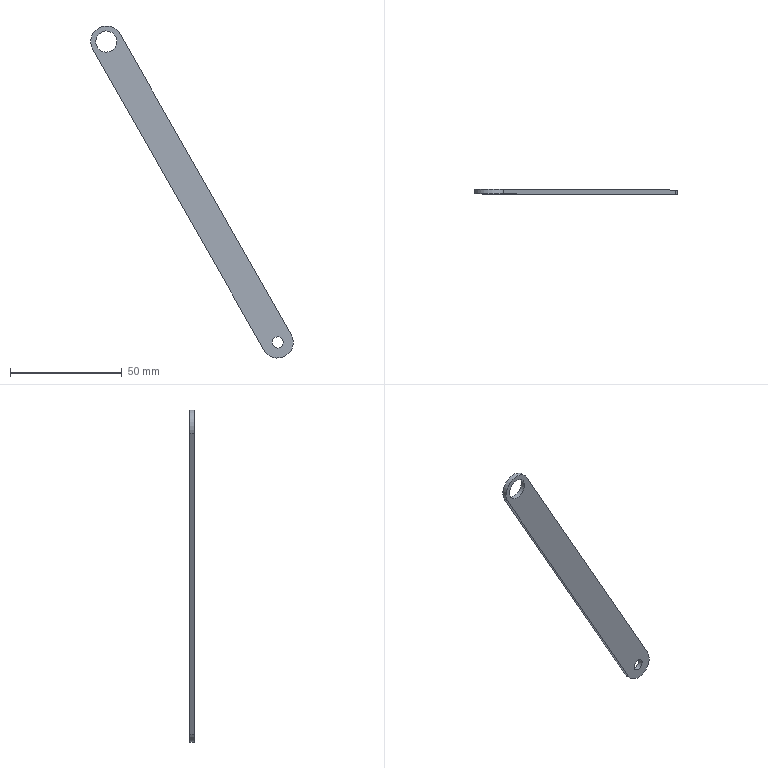Component | NX | 8 | 1 solid | 8 faces | box 90.7 x 2 x 148.69 mm | volume 4467 mm3 | cylinder 4 | plane 4 | commonest cylinder face diameters 14 x2 5 x1 9.5 x1
STEP:
#1=CARTESIAN_POINT('',(0.,0.,0.));
#2=DIRECTION('',(0.,0.,1.));
#3=DIRECTION('',(1.,0.,0.));
#4=AXIS2_PLACEMENT_3D('',#1,#2,#3);
#5=CARTESIAN_POINT('',(-289.091,186.249,-214.872));
#6=VERTEX_POINT('',#5);
#7=CARTESIAN_POINT('',(-276.925,186.249,-207.944));
#8=VERTEX_POINT('',#7);
#9=CARTESIAN_POINT('',(-283.008,186.249,-211.408));
#10=DIRECTION('',(0.,-1.,0.));
#11=DIRECTION('',(0.4948,0.,-0.869));
#12=AXIS2_PLACEMENT_3D('',#9,#10,#11);
#13=CIRCLE('',#12,7.);
#14=CARTESIAN_POINT('',(-283.008,184.249,-211.408));
#15=DIRECTION('',(0.,1.,0.));
#16=DIRECTION('',(0.4948,0.,-0.869));
#17=AXIS2_PLACEMENT_3D('',#14,#15,#16);
#18=CYLINDRICAL_SURFACE('',#17,7.);
#19=CARTESIAN_POINT('',(6.283,2.));
#20=DIRECTION('',(-1.,0.));
#21=VECTOR('',#20,1.);
#22=LINE('',#19,#21);
#23=(GEOMETRIC_REPRESENTATION_CONTEXT(2)PARAMETRIC_REPRESENTATION_CONTEXT()REPRESENTATION_CONTEXT('',''));
#24=DEFINITIONAL_REPRESENTATION('',(#22),#23);
#25=PCURVE('',#18,#24);
#26=CARTESIAN_POINT('',(-283.008,186.249,-211.408));
#27=DIRECTION('',(0.,-1.,0.));
#28=DIRECTION('',(-0.4948,0.,0.869));
#29=AXIS2_PLACEMENT_3D('',#26,#27,#28);
#30=PLANE('',#29);
#31=CARTESIAN_POINT('',(0.,0.));
#32=DIRECTION('',(-1.,0.));
#33=AXIS2_PLACEMENT_2D('',#31,#32);
#34=CIRCLE('',#33,7.);
#35=(GEOMETRIC_REPRESENTATION_CONTEXT(2)PARAMETRIC_REPRESENTATION_CONTEXT()REPRESENTATION_CONTEXT('',''));
#36=DEFINITIONAL_REPRESENTATION('',(#34),#35);
#37=PCURVE('',#30,#36);
#38=SURFACE_CURVE('',#13,(#25,#37),.PCURVE_S1.);
#39=EDGE_CURVE('',#6,#8,#38,.T.);
#40=ORIENTED_EDGE('',*,*,#39,.T.);
#41=CARTESIAN_POINT('',(-276.925,184.249,-207.944));
#42=VERTEX_POINT('',#41);
#43=CARTESIAN_POINT('',(-276.925,184.249,-207.944));
#44=DIRECTION('',(0.,1.,0.));
#45=VECTOR('',#44,1.);
#46=LINE('',#43,#45);
#47=CARTESIAN_POINT('',(-1.571,0.));
#48=DIRECTION('',(0.,1.));
#49=VECTOR('',#48,1.);
#50=LINE('',#47,#49);
#51=(GEOMETRIC_REPRESENTATION_CONTEXT(2)PARAMETRIC_REPRESENTATION_CONTEXT()REPRESENTATION_CONTEXT('',''));
#52=DEFINITIONAL_REPRESENTATION('',(#50),#51);
#53=PCURVE('',#18,#52);
#54=CARTESIAN_POINT('',(-276.925,184.249,-207.944));
#55=DIRECTION('',(-0.869,0.,-0.4948));
#56=DIRECTION('',(0.,-1.,0.));
#57=AXIS2_PLACEMENT_3D('',#54,#55,#56);
#58=PLANE('',#57);
#59=CARTESIAN_POINT('',(0.,-0.));
#60=DIRECTION('',(-1.,0.));
#61=VECTOR('',#60,1.);
#62=LINE('',#59,#61);
#63=(GEOMETRIC_REPRESENTATION_CONTEXT(2)PARAMETRIC_REPRESENTATION_CONTEXT()REPRESENTATION_CONTEXT('',''));
#64=DEFINITIONAL_REPRESENTATION('',(#62),#63);
#65=PCURVE('',#58,#64);
#66=SURFACE_CURVE('',#46,(#53,#65),.PCURVE_S1.);
#67=EDGE_CURVE('',#42,#8,#66,.T.);
#68=ORIENTED_EDGE('',*,*,#67,.F.);
#69=CARTESIAN_POINT('',(-289.091,184.249,-214.872));
#70=VERTEX_POINT('',#69);
#71=CARTESIAN_POINT('',(-283.008,184.249,-211.408));
#72=DIRECTION('',(0.,-1.,0.));
#73=DIRECTION('',(0.4948,0.,-0.869));
#74=AXIS2_PLACEMENT_3D('',#71,#72,#73);
#75=CIRCLE('',#74,7.);
#76=CARTESIAN_POINT('',(6.283,0.));
#77=DIRECTION('',(-1.,0.));
#78=VECTOR('',#77,1.);
#79=LINE('',#76,#78);
#80=(GEOMETRIC_REPRESENTATION_CONTEXT(2)PARAMETRIC_REPRESENTATION_CONTEXT()REPRESENTATION_CONTEXT('',''));
#81=DEFINITIONAL_REPRESENTATION('',(#79),#80);
#82=PCURVE('',#18,#81);
#83=CARTESIAN_POINT('',(-283.008,184.249,-211.408));
#84=DIRECTION('',(0.,-1.,0.));
#85=DIRECTION('',(-0.4948,0.,0.869));
#86=AXIS2_PLACEMENT_3D('',#83,#84,#85);
#87=PLANE('',#86);
#88=CARTESIAN_POINT('',(0.,0.));
#89=DIRECTION('',(-1.,0.));
#90=AXIS2_PLACEMENT_2D('',#88,#89);
#91=CIRCLE('',#90,7.);
#92=(GEOMETRIC_REPRESENTATION_CONTEXT(2)PARAMETRIC_REPRESENTATION_CONTEXT()REPRESENTATION_CONTEXT('',''));
#93=DEFINITIONAL_REPRESENTATION('',(#91),#92);
#94=PCURVE('',#87,#93);
#95=SURFACE_CURVE('',#75,(#82,#94),.PCURVE_S1.);
#96=EDGE_CURVE('',#70,#42,#95,.T.);
#97=ORIENTED_EDGE('',*,*,#96,.F.);
#98=CARTESIAN_POINT('',(-289.091,184.249,-214.872));
#99=DIRECTION('',(0.,1.,0.));
#100=VECTOR('',#99,1.);
#101=LINE('',#98,#100);
#102=CARTESIAN_POINT('',(1.571,0.));
#103=DIRECTION('',(0.,1.));
#104=VECTOR('',#103,1.);
#105=LINE('',#102,#104);
#106=(GEOMETRIC_REPRESENTATION_CONTEXT(2)PARAMETRIC_REPRESENTATION_CONTEXT()REPRESENTATION_CONTEXT('',''));
#107=DEFINITIONAL_REPRESENTATION('',(#105),#106);
#108=PCURVE('',#18,#107);
#109=CARTESIAN_POINT('',(-365.788,184.249,-80.178));
#110=DIRECTION('',(0.869,0.,0.4948));
#111=DIRECTION('',(0.,1.,0.));
#112=AXIS2_PLACEMENT_3D('',#109,#110,#111);
#113=PLANE('',#112);
#114=CARTESIAN_POINT('',(0.,-155.));
#115=DIRECTION('',(1.,0.));
#116=VECTOR('',#115,1.);
#117=LINE('',#114,#116);
#118=(GEOMETRIC_REPRESENTATION_CONTEXT(2)PARAMETRIC_REPRESENTATION_CONTEXT()REPRESENTATION_CONTEXT('',''));
#119=DEFINITIONAL_REPRESENTATION('',(#117),#118);
#120=PCURVE('',#113,#119);
#121=SURFACE_CURVE('',#101,(#108,#120),.PCURVE_S1.);
#122=EDGE_CURVE('',#70,#6,#121,.T.);
#123=ORIENTED_EDGE('',*,*,#122,.T.);
#124=EDGE_LOOP('',(#40,#68,#97,#123));
#125=FACE_BOUND('',#124,.T.);
#126=ADVANCED_FACE('',(#125),#18,.T.);
#127=CARTESIAN_POINT('',(-353.622,186.249,-73.25));
#128=VERTEX_POINT('',#127);
#129=CARTESIAN_POINT('',(-276.925,186.249,-207.944));
#130=DIRECTION('',(-0.4948,0.,0.869));
#131=VECTOR('',#130,1.);
#132=LINE('',#129,#131);
#133=CARTESIAN_POINT('',(-2.,0.));
#134=DIRECTION('',(0.,1.));
#135=VECTOR('',#134,1.);
#136=LINE('',#133,#135);
#137=(GEOMETRIC_REPRESENTATION_CONTEXT(2)PARAMETRIC_REPRESENTATION_CONTEXT()REPRESENTATION_CONTEXT('',''));
#138=DEFINITIONAL_REPRESENTATION('',(#136),#137);
#139=PCURVE('',#58,#138);
#140=CARTESIAN_POINT('',(0.,-7.));
#141=DIRECTION('',(1.,0.));
#142=VECTOR('',#141,1.);
#143=LINE('',#140,#142);
#144=(GEOMETRIC_REPRESENTATION_CONTEXT(2)PARAMETRIC_REPRESENTATION_CONTEXT()REPRESENTATION_CONTEXT('',''));
#145=DEFINITIONAL_REPRESENTATION('',(#143),#144);
#146=PCURVE('',#30,#145);
#147=SURFACE_CURVE('',#132,(#139,#146),.PCURVE_S1.);
#148=EDGE_CURVE('',#8,#128,#147,.T.);
#149=ORIENTED_EDGE('',*,*,#148,.T.);
#150=CARTESIAN_POINT('',(-353.622,184.249,-73.25));
#151=VERTEX_POINT('',#150);
#152=CARTESIAN_POINT('',(-353.622,184.249,-73.25));
#153=DIRECTION('',(0.,1.,0.));
#154=VECTOR('',#153,1.);
#155=LINE('',#152,#154);
#156=CARTESIAN_POINT('',(0.,155.));
#157=DIRECTION('',(-1.,0.));
#158=VECTOR('',#157,1.);
#159=LINE('',#156,#158);
#160=(GEOMETRIC_REPRESENTATION_CONTEXT(2)PARAMETRIC_REPRESENTATION_CONTEXT()REPRESENTATION_CONTEXT('',''));
#161=DEFINITIONAL_REPRESENTATION('',(#159),#160);
#162=PCURVE('',#58,#161);
#163=CARTESIAN_POINT('',(-359.705,184.249,-76.714));
#164=DIRECTION('',(0.,1.,0.));
#165=DIRECTION('',(0.4948,0.,-0.869));
#166=AXIS2_PLACEMENT_3D('',#163,#164,#165);
#167=CYLINDRICAL_SURFACE('',#166,7.);
#168=CARTESIAN_POINT('',(4.712,0.));
#169=DIRECTION('',(0.,1.));
#170=VECTOR('',#169,1.);
#171=LINE('',#168,#170);
#172=(GEOMETRIC_REPRESENTATION_CONTEXT(2)PARAMETRIC_REPRESENTATION_CONTEXT()REPRESENTATION_CONTEXT('',''));
#173=DEFINITIONAL_REPRESENTATION('',(#171),#172);
#174=PCURVE('',#167,#173);
#175=SURFACE_CURVE('',#155,(#162,#174),.PCURVE_S1.);
#176=EDGE_CURVE('',#151,#128,#175,.T.);
#177=ORIENTED_EDGE('',*,*,#176,.F.);
#178=CARTESIAN_POINT('',(-276.925,184.249,-207.944));
#179=DIRECTION('',(-0.4948,0.,0.869));
#180=VECTOR('',#179,1.);
#181=LINE('',#178,#180);
#182=CARTESIAN_POINT('',(0.,0.));
#183=DIRECTION('',(0.,1.));
#184=VECTOR('',#183,1.);
#185=LINE('',#182,#184);
#186=(GEOMETRIC_REPRESENTATION_CONTEXT(2)PARAMETRIC_REPRESENTATION_CONTEXT()REPRESENTATION_CONTEXT('',''));
#187=DEFINITIONAL_REPRESENTATION('',(#185),#186);
#188=PCURVE('',#58,#187);
#189=CARTESIAN_POINT('',(0.,-7.));
#190=DIRECTION('',(1.,0.));
#191=VECTOR('',#190,1.);
#192=LINE('',#189,#191);
#193=(GEOMETRIC_REPRESENTATION_CONTEXT(2)PARAMETRIC_REPRESENTATION_CONTEXT()REPRESENTATION_CONTEXT('',''));
#194=DEFINITIONAL_REPRESENTATION('',(#192),#193);
#195=PCURVE('',#87,#194);
#196=SURFACE_CURVE('',#181,(#188,#195),.PCURVE_S1.);
#197=EDGE_CURVE('',#42,#151,#196,.T.);
#198=ORIENTED_EDGE('',*,*,#197,.F.);
#199=ORIENTED_EDGE('',*,*,#67,.T.);
#200=EDGE_LOOP('',(#149,#177,#198,#199));
#201=FACE_BOUND('',#200,.T.);
#202=ADVANCED_FACE('',(#201),#58,.F.);
#203=CARTESIAN_POINT('',(-365.788,186.249,-80.178));
#204=VERTEX_POINT('',#203);
#205=CARTESIAN_POINT('',(-359.705,186.249,-76.714));
#206=DIRECTION('',(0.,-1.,0.));
#207=DIRECTION('',(0.4948,0.,-0.869));
#208=AXIS2_PLACEMENT_3D('',#205,#206,#207);
#209=CIRCLE('',#208,7.);
#210=CARTESIAN_POINT('',(6.283,2.));
#211=DIRECTION('',(-1.,0.));
#212=VECTOR('',#211,1.);
#213=LINE('',#210,#212);
#214=(GEOMETRIC_REPRESENTATION_CONTEXT(2)PARAMETRIC_REPRESENTATION_CONTEXT()REPRESENTATION_CONTEXT('',''));
#215=DEFINITIONAL_REPRESENTATION('',(#213),#214);
#216=PCURVE('',#167,#215);
#217=CARTESIAN_POINT('',(155.,0.));
#218=DIRECTION('',(-1.,-0.));
#219=AXIS2_PLACEMENT_2D('',#217,#218);
#220=CIRCLE('',#219,7.);
#221=(GEOMETRIC_REPRESENTATION_CONTEXT(2)PARAMETRIC_REPRESENTATION_CONTEXT()REPRESENTATION_CONTEXT('',''));
#222=DEFINITIONAL_REPRESENTATION('',(#220),#221);
#223=PCURVE('',#30,#222);
#224=SURFACE_CURVE('',#209,(#216,#223),.PCURVE_S1.);
#225=EDGE_CURVE('',#128,#204,#224,.T.);
#226=ORIENTED_EDGE('',*,*,#225,.T.);
#227=CARTESIAN_POINT('',(-365.788,184.249,-80.178));
#228=VERTEX_POINT('',#227);
#229=CARTESIAN_POINT('',(-365.788,184.249,-80.178));
#230=DIRECTION('',(0.,1.,0.));
#231=VECTOR('',#230,1.);
#232=LINE('',#229,#231);
#233=CARTESIAN_POINT('',(1.571,0.));
#234=DIRECTION('',(0.,1.));
#235=VECTOR('',#234,1.);
#236=LINE('',#233,#235);
#237=(GEOMETRIC_REPRESENTATION_CONTEXT(2)PARAMETRIC_REPRESENTATION_CONTEXT()REPRESENTATION_CONTEXT('',''));
#238=DEFINITIONAL_REPRESENTATION('',(#236),#237);
#239=PCURVE('',#167,#238);
#240=CARTESIAN_POINT('',(0.,0.));
#241=DIRECTION('',(1.,0.));
#242=VECTOR('',#241,1.);
#243=LINE('',#240,#242);
#244=(GEOMETRIC_REPRESENTATION_CONTEXT(2)PARAMETRIC_REPRESENTATION_CONTEXT()REPRESENTATION_CONTEXT('',''));
#245=DEFINITIONAL_REPRESENTATION('',(#243),#244);
#246=PCURVE('',#113,#245);
#247=SURFACE_CURVE('',#232,(#239,#246),.PCURVE_S1.);
#248=EDGE_CURVE('',#228,#204,#247,.T.);
#249=ORIENTED_EDGE('',*,*,#248,.F.);
#250=CARTESIAN_POINT('',(-359.705,184.249,-76.714));
#251=DIRECTION('',(0.,-1.,0.));
#252=DIRECTION('',(0.4948,0.,-0.869));
#253=AXIS2_PLACEMENT_3D('',#250,#251,#252);
#254=CIRCLE('',#253,7.);
#255=CARTESIAN_POINT('',(6.283,0.));
#256=DIRECTION('',(-1.,0.));
#257=VECTOR('',#256,1.);
#258=LINE('',#255,#257);
#259=(GEOMETRIC_REPRESENTATION_CONTEXT(2)PARAMETRIC_REPRESENTATION_CONTEXT()REPRESENTATION_CONTEXT('',''));
#260=DEFINITIONAL_REPRESENTATION('',(#258),#259);
#261=PCURVE('',#167,#260);
#262=CARTESIAN_POINT('',(155.,0.));
#263=DIRECTION('',(-1.,-0.));
#264=AXIS2_PLACEMENT_2D('',#262,#263);
#265=CIRCLE('',#264,7.);
#266=(GEOMETRIC_REPRESENTATION_CONTEXT(2)PARAMETRIC_REPRESENTATION_CONTEXT()REPRESENTATION_CONTEXT('',''));
#267=DEFINITIONAL_REPRESENTATION('',(#265),#266);
#268=PCURVE('',#87,#267);
#269=SURFACE_CURVE('',#254,(#261,#268),.PCURVE_S1.);
#270=EDGE_CURVE('',#151,#228,#269,.T.);
#271=ORIENTED_EDGE('',*,*,#270,.F.);
#272=ORIENTED_EDGE('',*,*,#176,.T.);
#273=EDGE_LOOP('',(#226,#249,#271,#272));
#274=FACE_BOUND('',#273,.T.);
#275=ADVANCED_FACE('',(#274),#167,.T.);
#276=CARTESIAN_POINT('',(-284.245,184.249,-209.236));
#277=VERTEX_POINT('',#276);
#278=CARTESIAN_POINT('',(-283.008,184.249,-211.408));
#279=DIRECTION('',(0.,-1.,0.));
#280=DIRECTION('',(-0.4948,0.,0.869));
#281=AXIS2_PLACEMENT_3D('',#278,#279,#280);
#282=CIRCLE('',#281,2.5);
#283=CARTESIAN_POINT('',(-283.008,184.249,-211.408));
#284=DIRECTION('',(0.,1.,0.));
#285=DIRECTION('',(0.4948,0.,-0.869));
#286=AXIS2_PLACEMENT_3D('',#283,#284,#285);
#287=CYLINDRICAL_SURFACE('',#286,2.5);
#288=CARTESIAN_POINT('',(9.425,0.));
#289=DIRECTION('',(-1.,0.));
#290=VECTOR('',#289,1.);
#291=LINE('',#288,#290);
#292=(GEOMETRIC_REPRESENTATION_CONTEXT(2)PARAMETRIC_REPRESENTATION_CONTEXT()REPRESENTATION_CONTEXT('',''));
#293=DEFINITIONAL_REPRESENTATION('',(#291),#292);
#294=PCURVE('',#287,#293);
#295=CARTESIAN_POINT('',(0.,0.));
#296=DIRECTION('',(1.,0.));
#297=AXIS2_PLACEMENT_2D('',#295,#296);
#298=CIRCLE('',#297,2.5);
#299=(GEOMETRIC_REPRESENTATION_CONTEXT(2)PARAMETRIC_REPRESENTATION_CONTEXT()REPRESENTATION_CONTEXT('',''));
#300=DEFINITIONAL_REPRESENTATION('',(#298),#299);
#301=PCURVE('',#87,#300);
#302=SURFACE_CURVE('',#282,(#294,#301),.PCURVE_S1.);
#303=EDGE_CURVE('',#277,#277,#302,.T.);
#304=ORIENTED_EDGE('',*,*,#303,.F.);
#305=CARTESIAN_POINT('',(-284.245,186.249,-209.236));
#306=VERTEX_POINT('',#305);
#307=CARTESIAN_POINT('',(-284.245,184.249,-209.236));
#308=CARTESIAN_POINT('',(-284.245,186.249,-209.236));
#309=B_SPLINE_CURVE_WITH_KNOTS('',1,(#307,#308),.UNSPECIFIED.,.F.,.F.,(2,2),(0.,2.),.PIECEWISE_BEZIER_KNOTS.);
#310=CARTESIAN_POINT('',(9.425,0.));
#311=DIRECTION('',(0.,1.));
#312=VECTOR('',#311,1.);
#313=LINE('',#310,#312);
#314=(GEOMETRIC_REPRESENTATION_CONTEXT(2)PARAMETRIC_REPRESENTATION_CONTEXT()REPRESENTATION_CONTEXT('',''));
#315=DEFINITIONAL_REPRESENTATION('',(#313),#314);
#316=PCURVE('',#287,#315);
#317=CARTESIAN_POINT('',(3.142,0.));
#318=DIRECTION('',(0.,1.));
#319=VECTOR('',#318,1.);
#320=LINE('',#317,#319);
#321=(GEOMETRIC_REPRESENTATION_CONTEXT(2)PARAMETRIC_REPRESENTATION_CONTEXT()REPRESENTATION_CONTEXT('',''));
#322=DEFINITIONAL_REPRESENTATION('',(#320),#321);
#323=PCURVE('',#287,#322);
#324=SEAM_CURVE('',#309,(#316,#323),.PCURVE_S1.);
#325=EDGE_CURVE('',#277,#306,#324,.T.);
#326=ORIENTED_EDGE('',*,*,#325,.T.);
#327=CARTESIAN_POINT('',(-283.008,186.249,-211.408));
#328=DIRECTION('',(0.,-1.,0.));
#329=DIRECTION('',(-0.4948,0.,0.869));
#330=AXIS2_PLACEMENT_3D('',#327,#328,#329);
#331=CIRCLE('',#330,2.5);
#332=CARTESIAN_POINT('',(9.425,2.));
#333=DIRECTION('',(-1.,0.));
#334=VECTOR('',#333,1.);
#335=LINE('',#332,#334);
#336=(GEOMETRIC_REPRESENTATION_CONTEXT(2)PARAMETRIC_REPRESENTATION_CONTEXT()REPRESENTATION_CONTEXT('',''));
#337=DEFINITIONAL_REPRESENTATION('',(#335),#336);
#338=PCURVE('',#287,#337);
#339=CARTESIAN_POINT('',(0.,0.));
#340=DIRECTION('',(1.,0.));
#341=AXIS2_PLACEMENT_2D('',#339,#340);
#342=CIRCLE('',#341,2.5);
#343=(GEOMETRIC_REPRESENTATION_CONTEXT(2)PARAMETRIC_REPRESENTATION_CONTEXT()REPRESENTATION_CONTEXT('',''));
#344=DEFINITIONAL_REPRESENTATION('',(#342),#343);
#345=PCURVE('',#30,#344);
#346=SURFACE_CURVE('',#331,(#338,#345),.PCURVE_S1.);
#347=EDGE_CURVE('',#306,#306,#346,.T.);
#348=ORIENTED_EDGE('',*,*,#347,.T.);
#349=ORIENTED_EDGE('',*,*,#325,.F.);
#350=EDGE_LOOP('',(#304,#326,#348,#349));
#351=FACE_BOUND('',#350,.F.);
#352=ADVANCED_FACE('',(#351),#287,.F.);
#353=CARTESIAN_POINT('',(-365.788,186.249,-80.178));
#354=DIRECTION('',(0.4948,0.,-0.869));
#355=VECTOR('',#354,1.);
#356=LINE('',#353,#355);
#357=CARTESIAN_POINT('',(2.,0.));
#358=DIRECTION('',(0.,-1.));
#359=VECTOR('',#358,1.);
#360=LINE('',#357,#359);
#361=(GEOMETRIC_REPRESENTATION_CONTEXT(2)PARAMETRIC_REPRESENTATION_CONTEXT()REPRESENTATION_CONTEXT('',''));
#362=DEFINITIONAL_REPRESENTATION('',(#360),#361);
#363=PCURVE('',#113,#362);
#364=CARTESIAN_POINT('',(155.,7.));
#365=DIRECTION('',(-1.,0.));
#366=VECTOR('',#365,1.);
#367=LINE('',#364,#366);
#368=(GEOMETRIC_REPRESENTATION_CONTEXT(2)PARAMETRIC_REPRESENTATION_CONTEXT()REPRESENTATION_CONTEXT('',''));
#369=DEFINITIONAL_REPRESENTATION('',(#367),#368);
#370=PCURVE('',#30,#369);
#371=SURFACE_CURVE('',#356,(#363,#370),.PCURVE_S1.);
#372=EDGE_CURVE('',#204,#6,#371,.T.);
#373=ORIENTED_EDGE('',*,*,#372,.T.);
#374=ORIENTED_EDGE('',*,*,#122,.F.);
#375=CARTESIAN_POINT('',(-365.788,184.249,-80.178));
#376=DIRECTION('',(0.4948,0.,-0.869));
#377=VECTOR('',#376,1.);
#378=LINE('',#375,#377);
#379=CARTESIAN_POINT('',(0.,0.));
#380=DIRECTION('',(0.,-1.));
#381=VECTOR('',#380,1.);
#382=LINE('',#379,#381);
#383=(GEOMETRIC_REPRESENTATION_CONTEXT(2)PARAMETRIC_REPRESENTATION_CONTEXT()REPRESENTATION_CONTEXT('',''));
#384=DEFINITIONAL_REPRESENTATION('',(#382),#383);
#385=PCURVE('',#113,#384);
#386=CARTESIAN_POINT('',(155.,7.));
#387=DIRECTION('',(-1.,0.));
#388=VECTOR('',#387,1.);
#389=LINE('',#386,#388);
#390=(GEOMETRIC_REPRESENTATION_CONTEXT(2)PARAMETRIC_REPRESENTATION_CONTEXT()REPRESENTATION_CONTEXT('',''));
#391=DEFINITIONAL_REPRESENTATION('',(#389),#390);
#392=PCURVE('',#87,#391);
#393=SURFACE_CURVE('',#378,(#385,#392),.PCURVE_S1.);
#394=EDGE_CURVE('',#228,#70,#393,.T.);
#395=ORIENTED_EDGE('',*,*,#394,.F.);
#396=ORIENTED_EDGE('',*,*,#248,.T.);
#397=EDGE_LOOP('',(#373,#374,#395,#396));
#398=FACE_BOUND('',#397,.T.);
#399=ADVANCED_FACE('',(#398),#113,.F.);
#400=CARTESIAN_POINT('',(-357.355,184.249,-80.842));
#401=VERTEX_POINT('',#400);
#402=CARTESIAN_POINT('',(-359.705,184.249,-76.714));
#403=DIRECTION('',(0.,-1.,0.));
#404=DIRECTION('',(0.4948,0.,-0.869));
#405=AXIS2_PLACEMENT_3D('',#402,#403,#404);
#406=CIRCLE('',#405,4.75);
#407=CARTESIAN_POINT('',(-359.705,184.249,-76.714));
#408=DIRECTION('',(0.,1.,0.));
#409=DIRECTION('',(0.4948,0.,-0.869));
#410=AXIS2_PLACEMENT_3D('',#407,#408,#409);
#411=CYLINDRICAL_SURFACE('',#410,4.75);
#412=CARTESIAN_POINT('',(6.283,0.));
#413=DIRECTION('',(-1.,0.));
#414=VECTOR('',#413,1.);
#415=LINE('',#412,#414);
#416=(GEOMETRIC_REPRESENTATION_CONTEXT(2)PARAMETRIC_REPRESENTATION_CONTEXT()REPRESENTATION_CONTEXT('',''));
#417=DEFINITIONAL_REPRESENTATION('',(#415),#416);
#418=PCURVE('',#411,#417);
#419=CARTESIAN_POINT('',(155.,0.));
#420=DIRECTION('',(-1.,0.));
#421=AXIS2_PLACEMENT_2D('',#419,#420);
#422=CIRCLE('',#421,4.75);
#423=(GEOMETRIC_REPRESENTATION_CONTEXT(2)PARAMETRIC_REPRESENTATION_CONTEXT()REPRESENTATION_CONTEXT('',''));
#424=DEFINITIONAL_REPRESENTATION('',(#422),#423);
#425=PCURVE('',#87,#424);
#426=SURFACE_CURVE('',#406,(#418,#425),.PCURVE_S1.);
#427=EDGE_CURVE('',#401,#401,#426,.T.);
#428=ORIENTED_EDGE('',*,*,#427,.F.);
#429=CARTESIAN_POINT('',(-357.355,186.249,-80.842));
#430=VERTEX_POINT('',#429);
#431=CARTESIAN_POINT('',(-357.355,184.249,-80.842));
#432=CARTESIAN_POINT('',(-357.355,186.249,-80.842));
#433=B_SPLINE_CURVE_WITH_KNOTS('',1,(#431,#432),.UNSPECIFIED.,.F.,.F.,(2,2),(0.,2.),.PIECEWISE_BEZIER_KNOTS.);
#434=CARTESIAN_POINT('',(6.283,0.));
#435=DIRECTION('',(0.,1.));
#436=VECTOR('',#435,1.);
#437=LINE('',#434,#436);
#438=(GEOMETRIC_REPRESENTATION_CONTEXT(2)PARAMETRIC_REPRESENTATION_CONTEXT()REPRESENTATION_CONTEXT('',''));
#439=DEFINITIONAL_REPRESENTATION('',(#437),#438);
#440=PCURVE('',#411,#439);
#441=CARTESIAN_POINT('',(0.,0.));
#442=DIRECTION('',(0.,1.));
#443=VECTOR('',#442,1.);
#444=LINE('',#441,#443);
#445=(GEOMETRIC_REPRESENTATION_CONTEXT(2)PARAMETRIC_REPRESENTATION_CONTEXT()REPRESENTATION_CONTEXT('',''));
#446=DEFINITIONAL_REPRESENTATION('',(#444),#445);
#447=PCURVE('',#411,#446);
#448=SEAM_CURVE('',#433,(#440,#447),.PCURVE_S1.);
#449=EDGE_CURVE('',#401,#430,#448,.T.);
#450=ORIENTED_EDGE('',*,*,#449,.T.);
#451=CARTESIAN_POINT('',(-359.705,186.249,-76.714));
#452=DIRECTION('',(0.,-1.,0.));
#453=DIRECTION('',(0.4948,0.,-0.869));
#454=AXIS2_PLACEMENT_3D('',#451,#452,#453);
#455=CIRCLE('',#454,4.75);
#456=CARTESIAN_POINT('',(6.283,2.));
#457=DIRECTION('',(-1.,0.));
#458=VECTOR('',#457,1.);
#459=LINE('',#456,#458);
#460=(GEOMETRIC_REPRESENTATION_CONTEXT(2)PARAMETRIC_REPRESENTATION_CONTEXT()REPRESENTATION_CONTEXT('',''));
#461=DEFINITIONAL_REPRESENTATION('',(#459),#460);
#462=PCURVE('',#411,#461);
#463=CARTESIAN_POINT('',(155.,0.));
#464=DIRECTION('',(-1.,0.));
#465=AXIS2_PLACEMENT_2D('',#463,#464);
#466=CIRCLE('',#465,4.75);
#467=(GEOMETRIC_REPRESENTATION_CONTEXT(2)PARAMETRIC_REPRESENTATION_CONTEXT()REPRESENTATION_CONTEXT('',''));
#468=DEFINITIONAL_REPRESENTATION('',(#466),#467);
#469=PCURVE('',#30,#468);
#470=SURFACE_CURVE('',#455,(#462,#469),.PCURVE_S1.);
#471=EDGE_CURVE('',#430,#430,#470,.T.);
#472=ORIENTED_EDGE('',*,*,#471,.T.);
#473=ORIENTED_EDGE('',*,*,#449,.F.);
#474=EDGE_LOOP('',(#428,#450,#472,#473));
#475=FACE_BOUND('',#474,.F.);
#476=ADVANCED_FACE('',(#475),#411,.F.);
#477=ORIENTED_EDGE('',*,*,#96,.T.);
#478=ORIENTED_EDGE('',*,*,#197,.T.);
#479=ORIENTED_EDGE('',*,*,#270,.T.);
#480=ORIENTED_EDGE('',*,*,#394,.T.);
#481=EDGE_LOOP('',(#477,#478,#479,#480));
#482=FACE_BOUND('',#481,.T.);
#483=ORIENTED_EDGE('',*,*,#303,.F.);
#484=EDGE_LOOP('',(#483));
#485=FACE_BOUND('',#484,.T.);
#486=ORIENTED_EDGE('',*,*,#427,.F.);
#487=EDGE_LOOP('',(#486));
#488=FACE_BOUND('',#487,.T.);
#489=ADVANCED_FACE('',(#482,#485,#488),#87,.T.);
#490=ORIENTED_EDGE('',*,*,#39,.F.);
#491=ORIENTED_EDGE('',*,*,#372,.F.);
#492=ORIENTED_EDGE('',*,*,#225,.F.);
#493=ORIENTED_EDGE('',*,*,#148,.F.);
#494=EDGE_LOOP('',(#490,#491,#492,#493));
#495=FACE_BOUND('',#494,.T.);
#496=ORIENTED_EDGE('',*,*,#347,.T.);
#497=EDGE_LOOP('',(#496));
#498=FACE_BOUND('',#497,.T.);
#499=ORIENTED_EDGE('',*,*,#471,.T.);
#500=EDGE_LOOP('',(#499));
#501=FACE_BOUND('',#500,.T.);
#502=ADVANCED_FACE('',(#495,#498,#501),#30,.F.);
#503=CLOSED_SHELL('',(#126,#202,#275,#352,#399,#476,#489,#502));
#504=MANIFOLD_SOLID_BREP('',#503);
#505=(LENGTH_UNIT()NAMED_UNIT(*)SI_UNIT(.MILLI.,.METRE.));
#506=UNCERTAINTY_MEASURE_WITH_UNIT(LENGTH_MEASURE(0.000002),#505,'','');
#507=(NAMED_UNIT(*)PLANE_ANGLE_UNIT()SI_UNIT($,.RADIAN.));
#508=(NAMED_UNIT(*)SI_UNIT($,.STERADIAN.)SOLID_ANGLE_UNIT());
#509=(GEOMETRIC_REPRESENTATION_CONTEXT(3)GLOBAL_UNCERTAINTY_ASSIGNED_CONTEXT((#506))GLOBAL_UNIT_ASSIGNED_CONTEXT((#505,#507,#508))REPRESENTATION_CONTEXT('',''));
#510=ADVANCED_BREP_SHAPE_REPRESENTATION('',(#4,#504),#509);